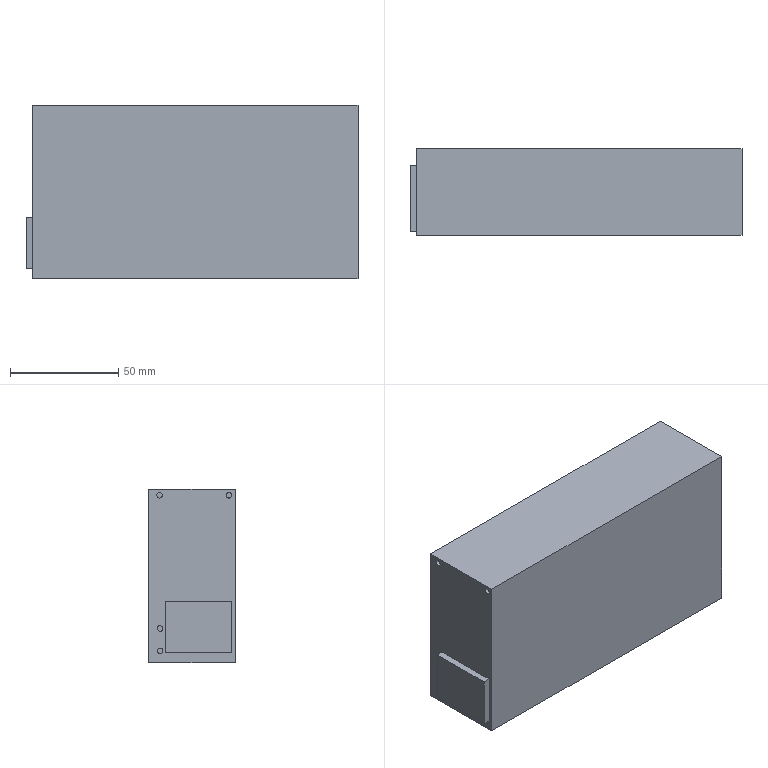Component | NX | POWER_SUPPLY | 1 solid | 19 faces | volume 481753 mm3 | plane 15 | cylinder 4 | commonest cylinder face diameters 2.61 x4